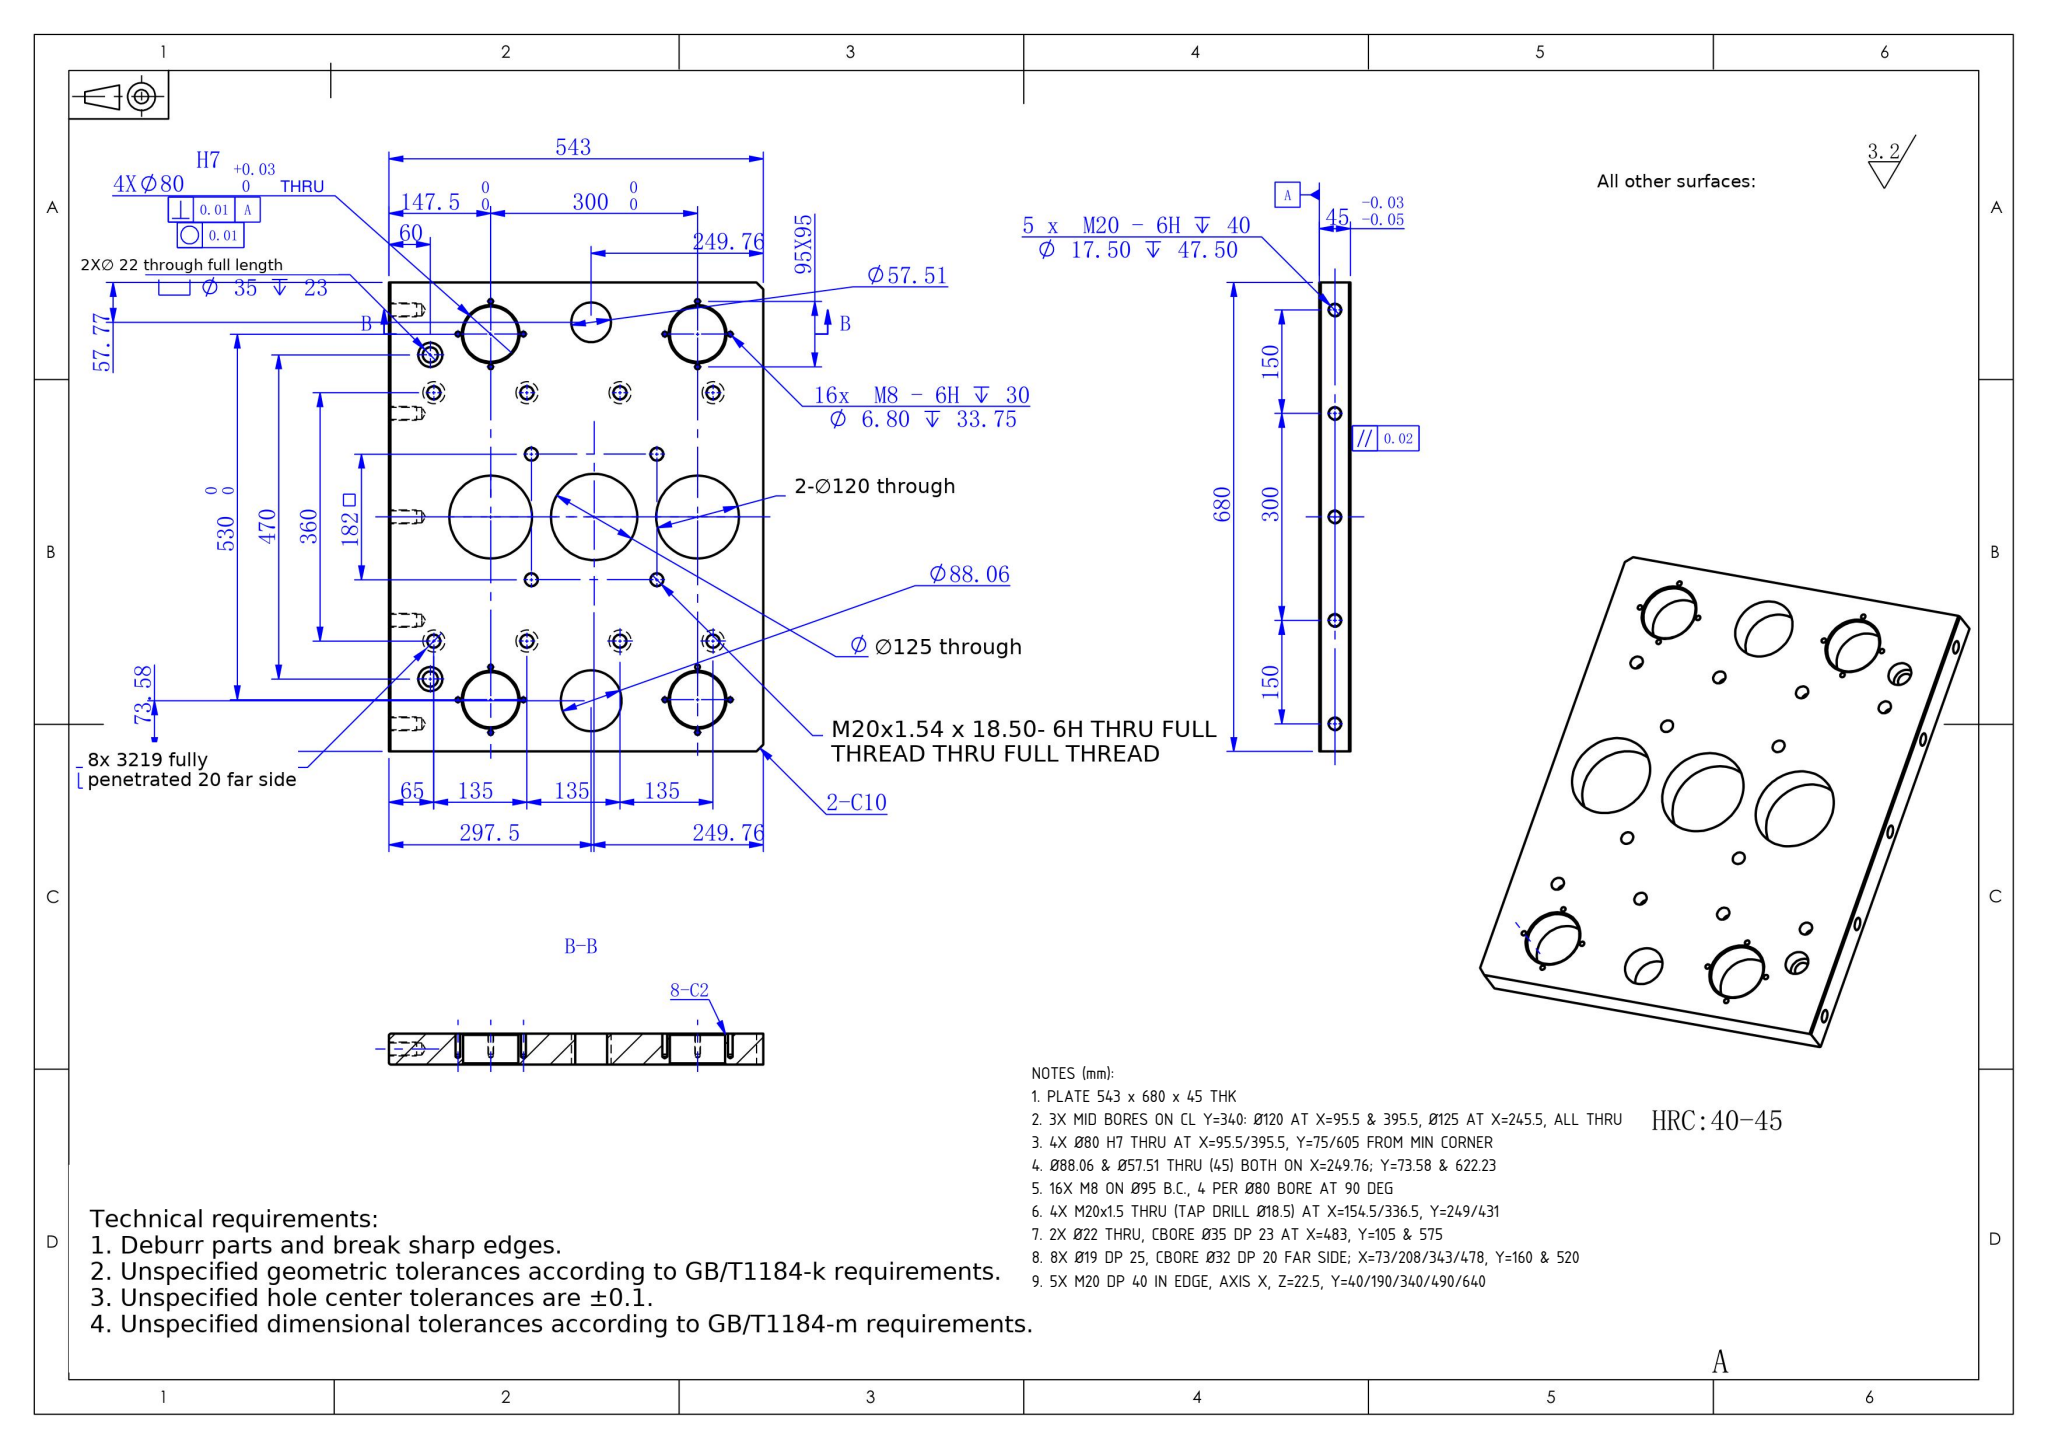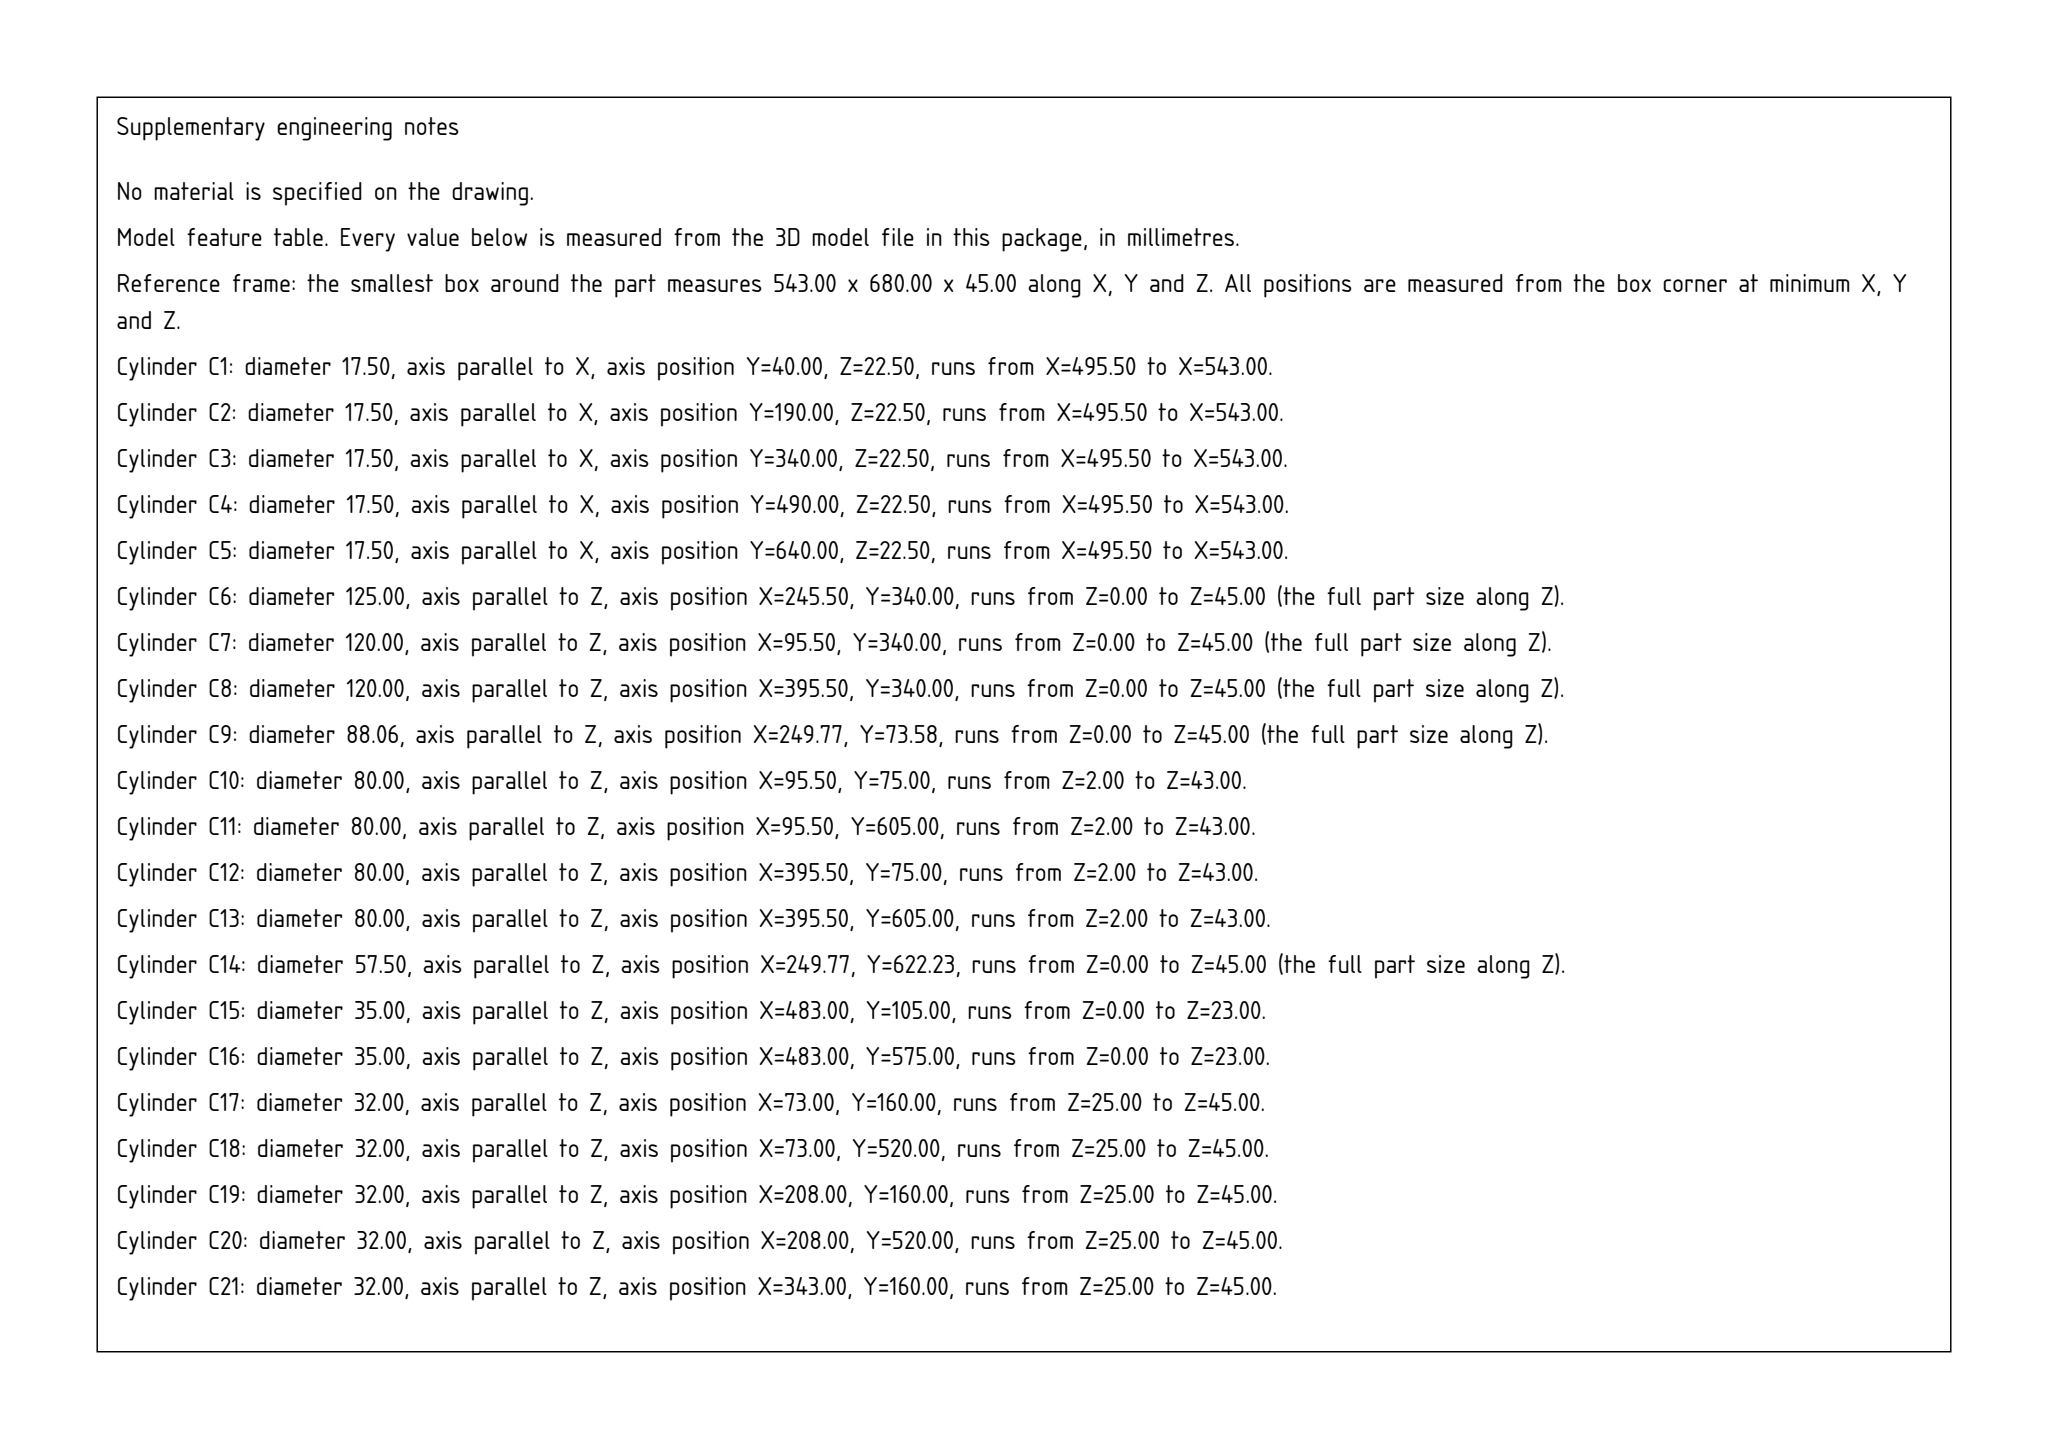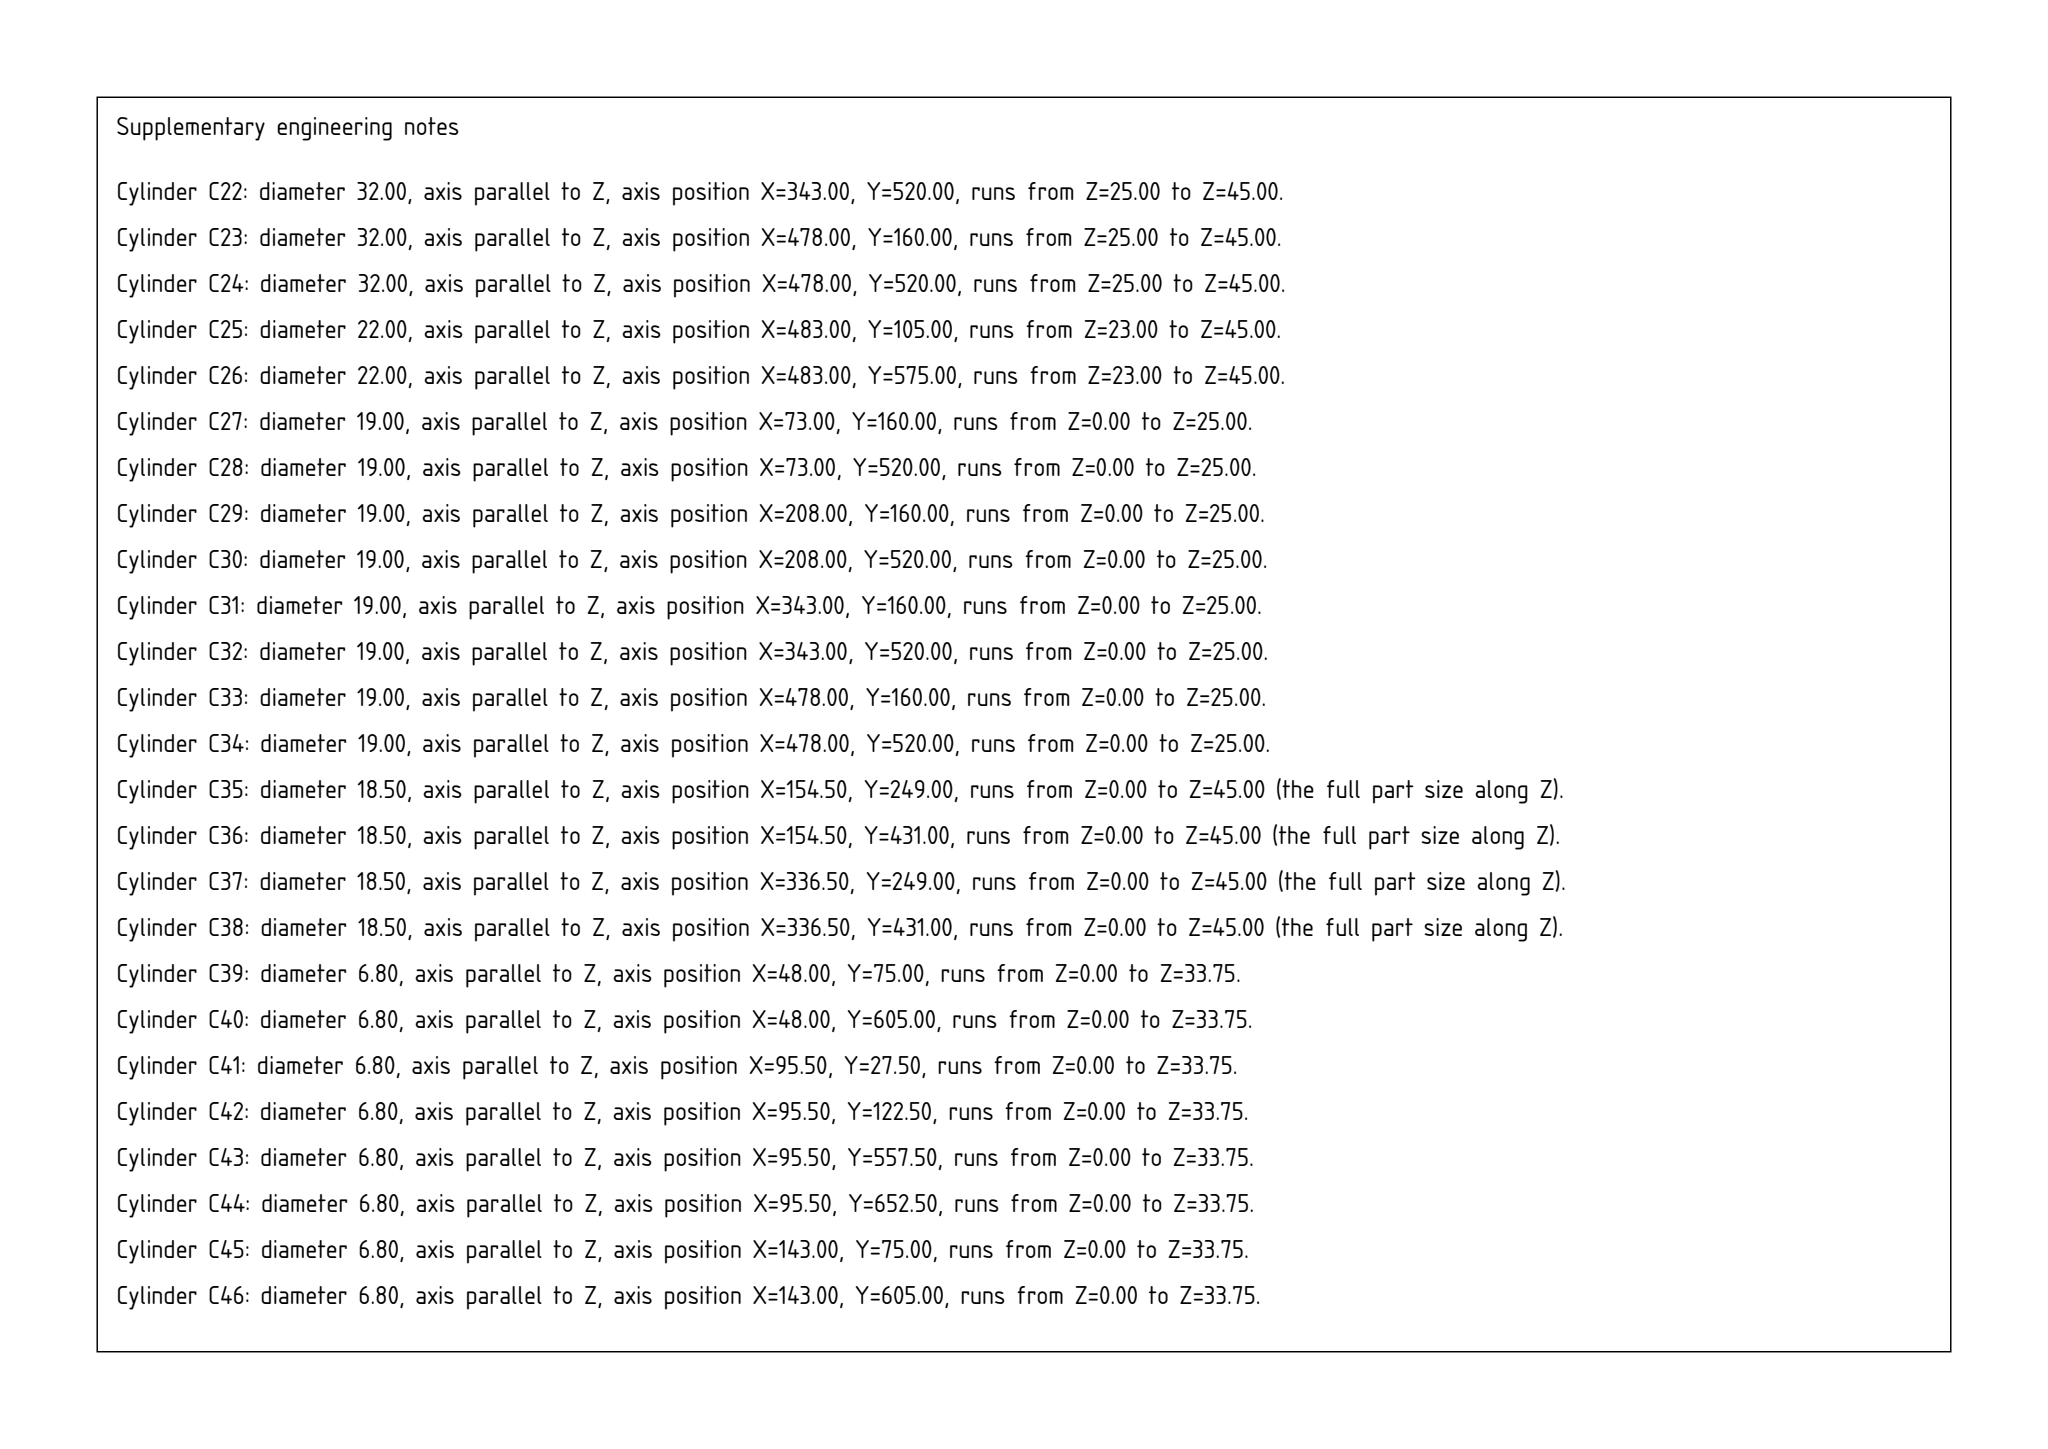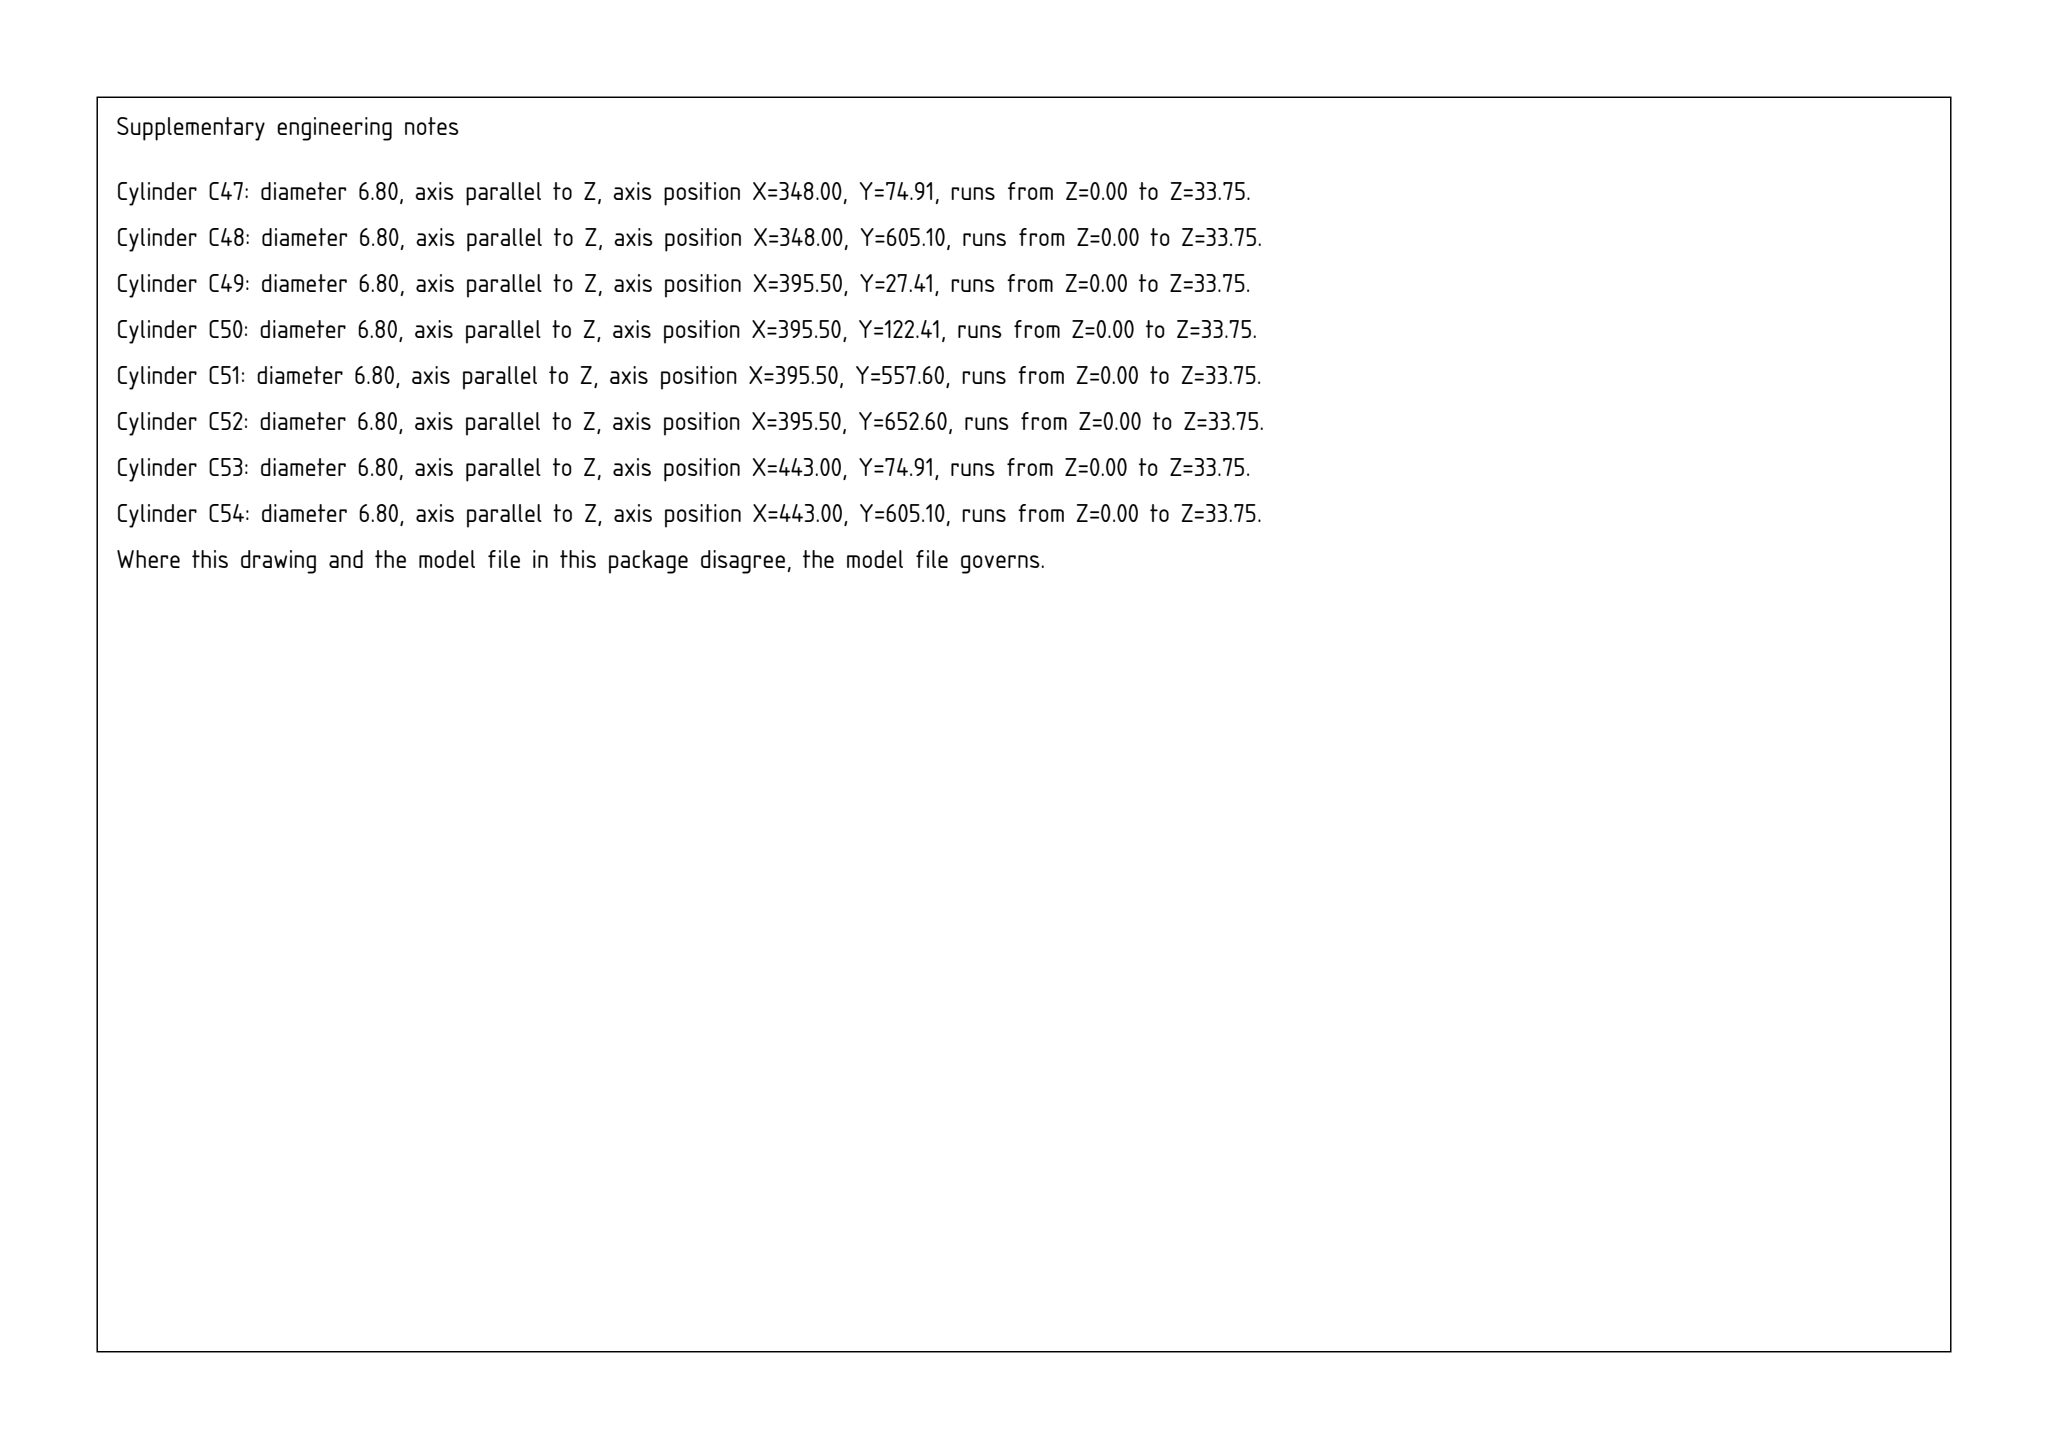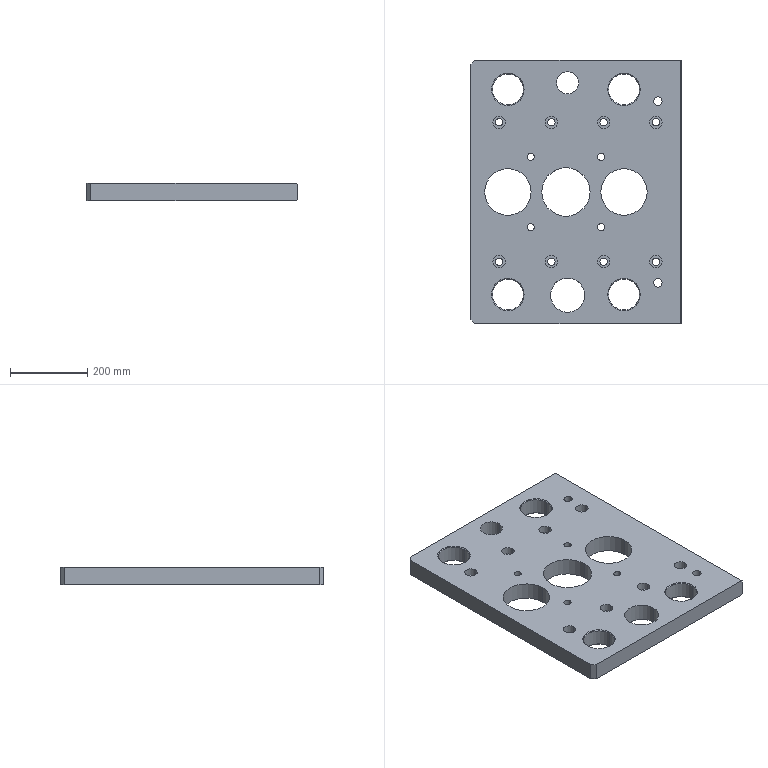Part | SolidWorks | mm | 1 solid | 186 faces | box 543 x 680 x 45 mm | volume 13364641 mm3 | cylinder 108 | cone 58 | plane 20 | commonest cylinder face diameters 6.8 x32 32 x16 19 x16 17.5 x10 80 x8 18.5 x8 35 x4 22 x4
Drawing notes:
PLATE 543 x 680 x 45 THK | from the solid: bbox_xyz 543,680,45
3X MID BORES ON CL Y=340: Ø120 AT X=95.5 & 395.5, Ø125 AT X=245.5, ALL THRU | from the solid: Ø120 z-cyls (95.5,340),(395.5,340) len 45; Ø125 (245.5,340) len 45
4X Ø80 H7 THRU AT X=95.5/395.5, Y=75/605 FROM MIN CORNER | from the solid: Ø80 z-cyls at (95.5,75),(95.5,605),(395.5,75),(395.5,605)
Ø88.06 & Ø57.51 THRU (45) BOTH ON X=249.76; Y=73.58 & 622.23 | from the solid: Ø88.06 at (249.76,73.58) len 45; Ø57.51 at (249.76,622.23) len 45
16X M8 ON Ø95 B.C., 4 PER Ø80 BORE AT 90 DEG | from the solid: Ø6.8 at (48,75),(95.5,27.5),(95.5,122.5),(143,75) about Ø80 ctr (95.5,75): R47.5
4X M20x1.5 THRU (TAP DRILL Ø18.5) AT X=154.5/336.5, Y=249/431 | from the solid: Ø18.5 z-cyls len 45 at (154.5,249),(154.5,431),(336.5,249),(336.5,431)
2X Ø22 THRU, CBORE Ø35 DP 23 AT X=483, Y=105 & 575 | from the solid: Ø22 len 22 at (483,105),(483,575); Ø35 len 23 same ctrs
8X Ø19 DP 25, CBORE Ø32 DP 20 FAR SIDE; X=73/208/343/478, Y=160 & 520 | from the solid: Ø19 len 25 and Ø32 len 20 pairs at X=73,208,343,478 with Y=160,520; z-plane 25 count 8
5X M20 DP 40 IN EDGE, AXIS X, Z=22.5, Y=40/190/340/490/640 | from the solid: Ø17.5 x-cyls len 47.5 at Y=40,190,340,490,640, Z=22.5